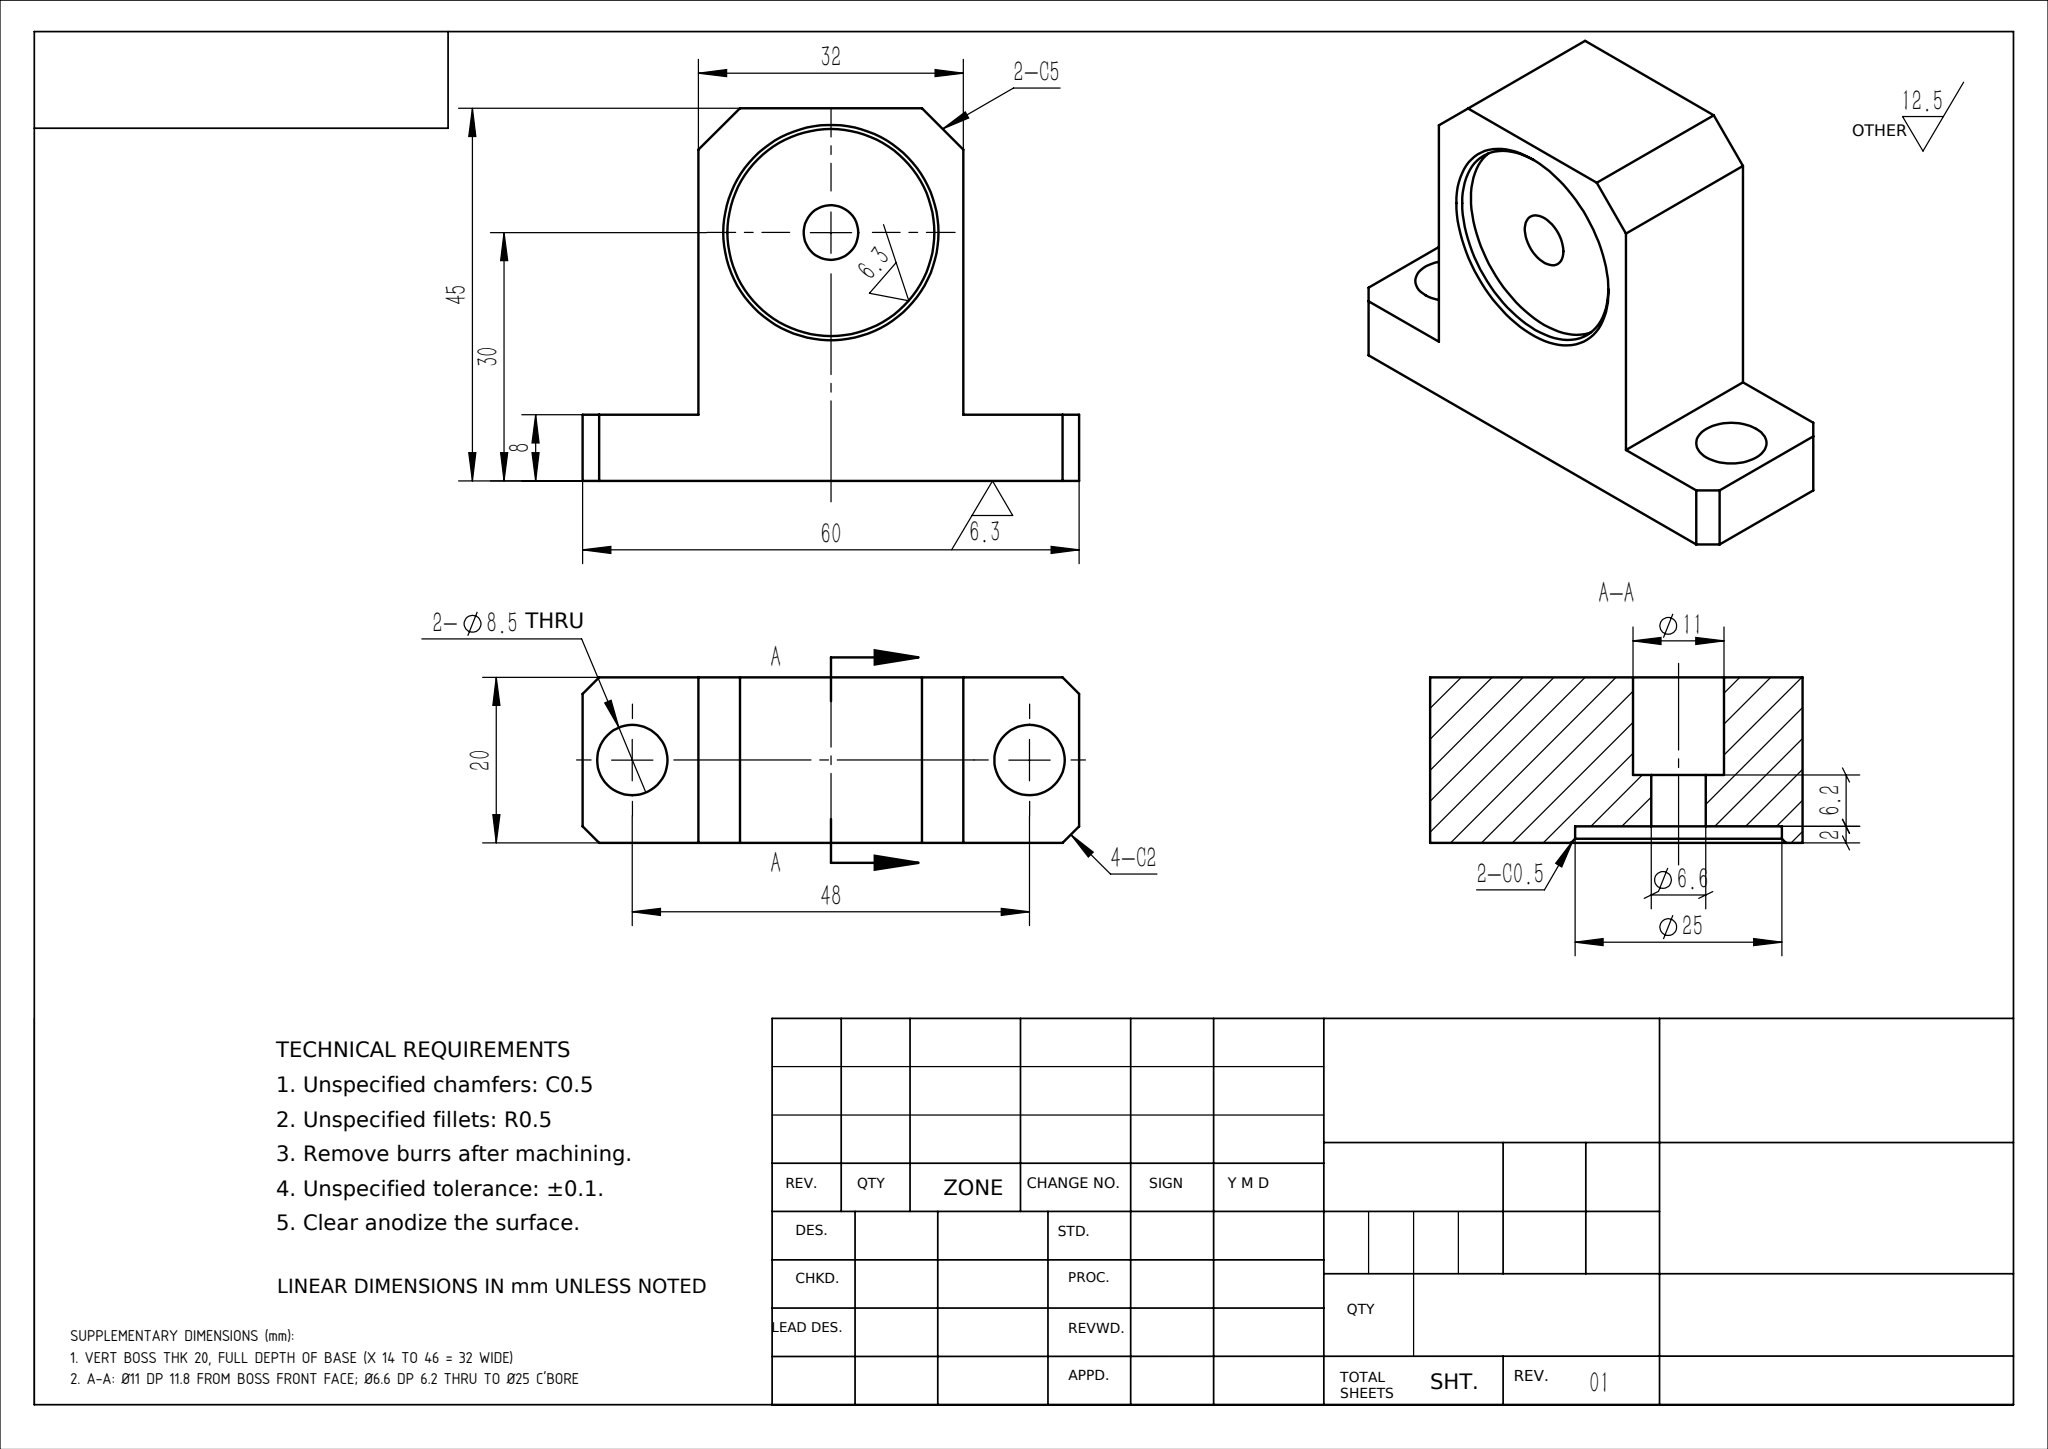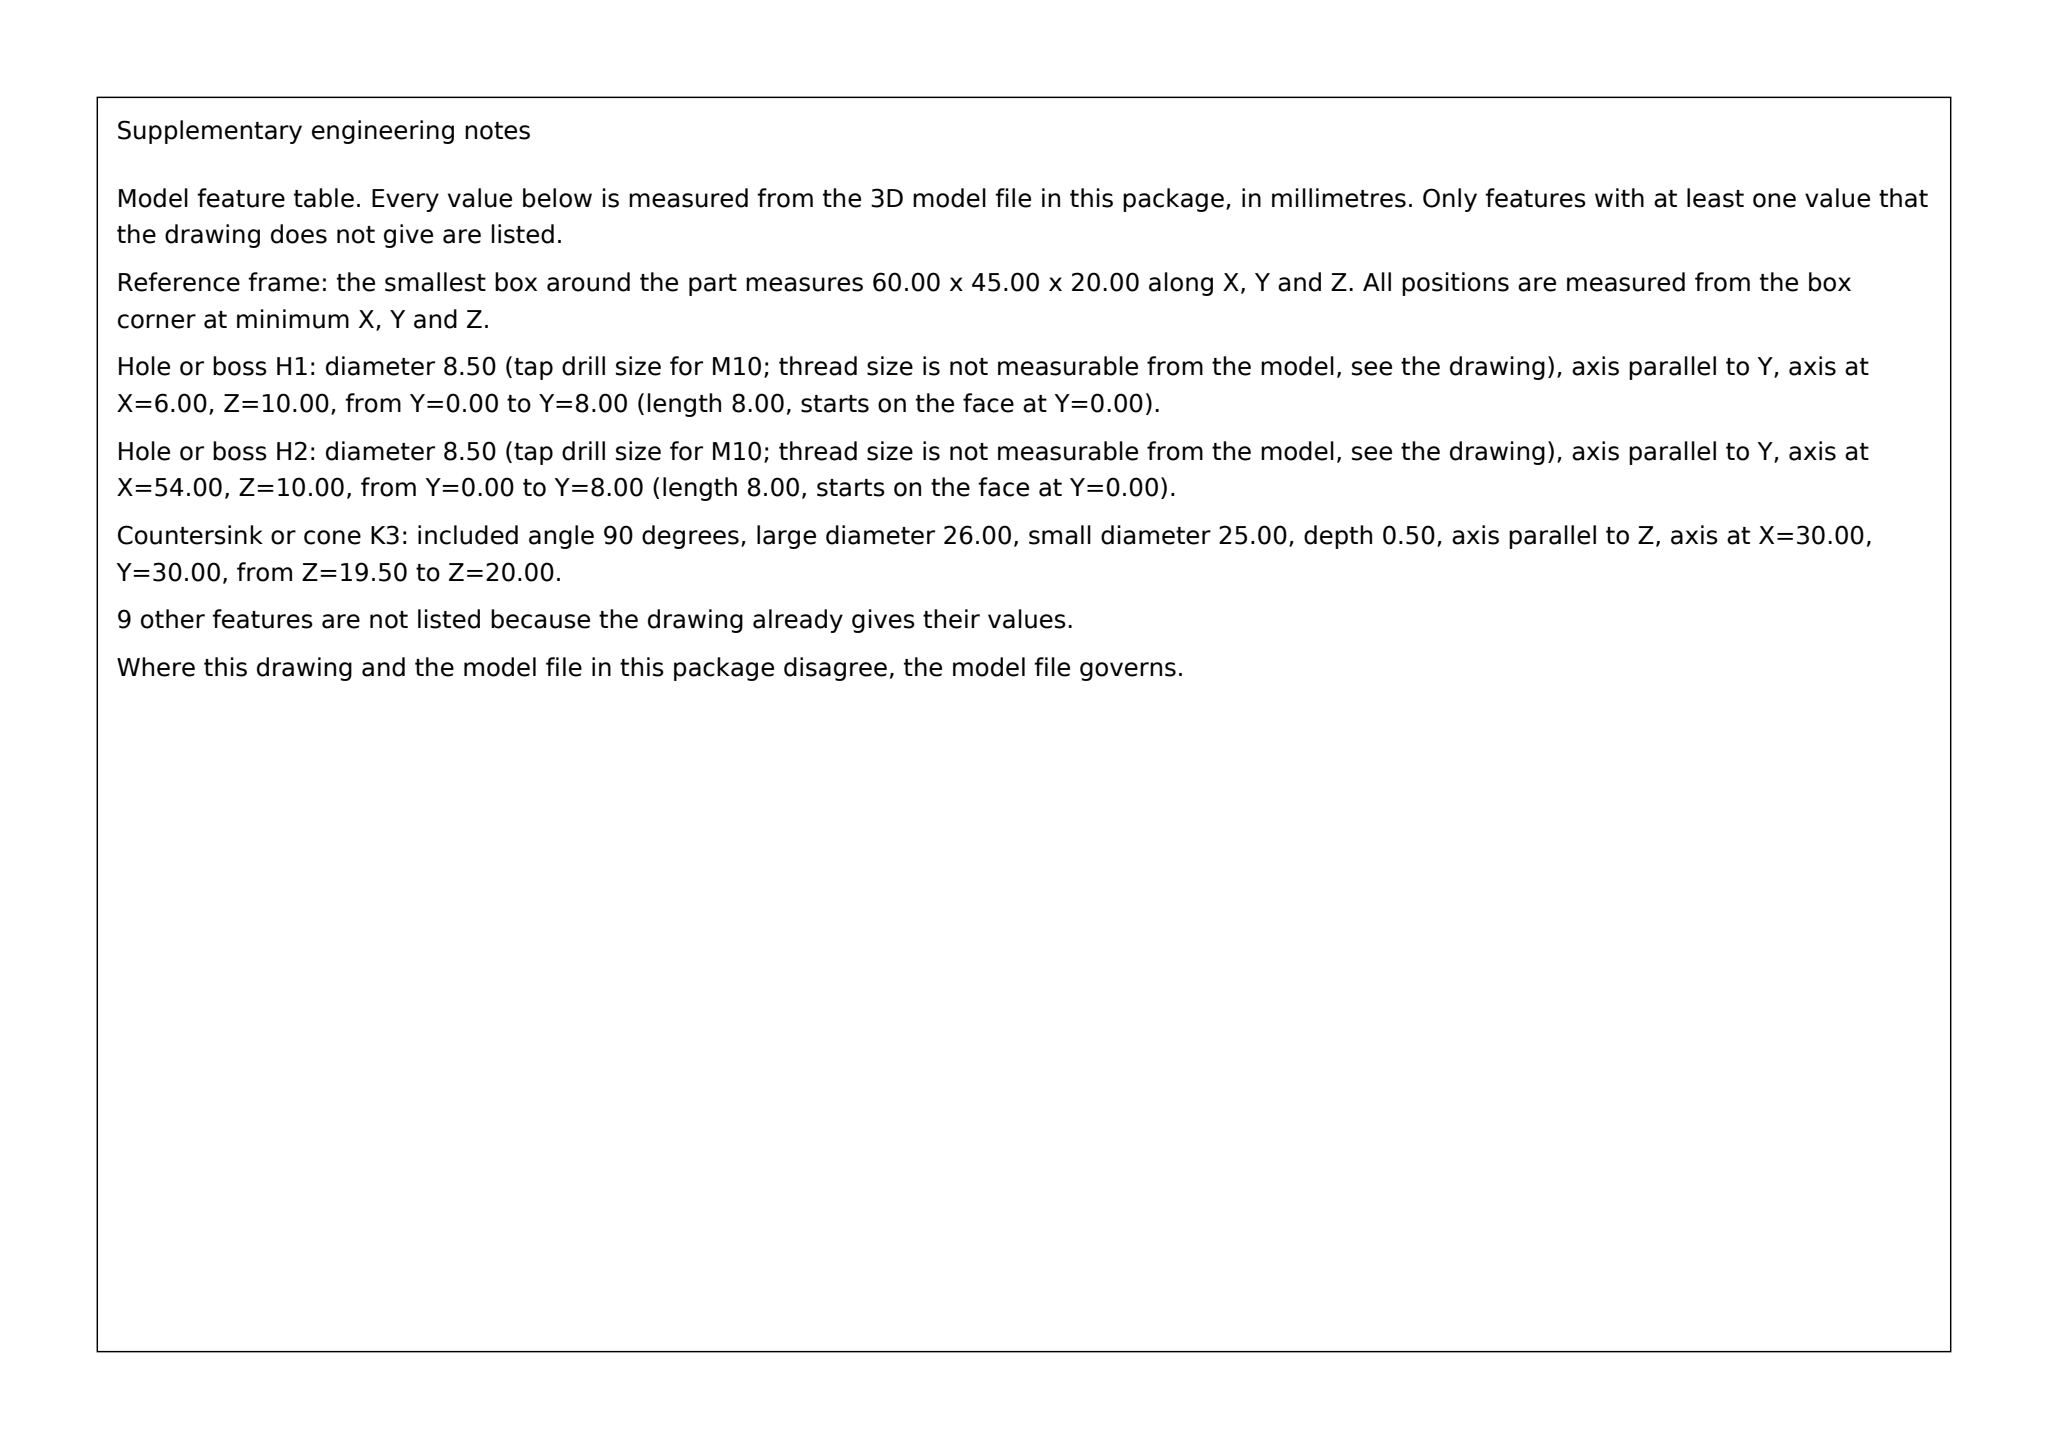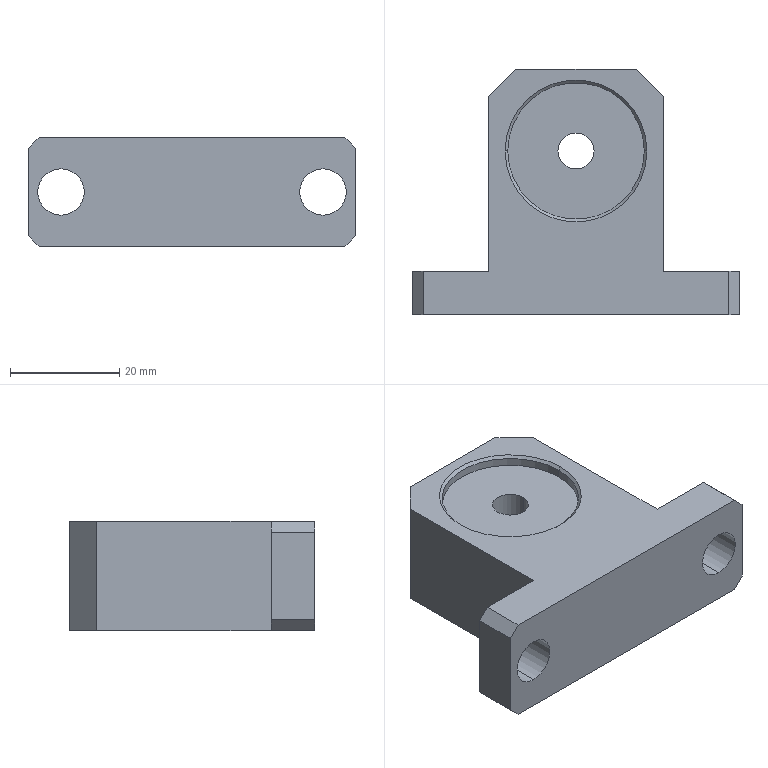Part | SolidWorks | mm | 1 solid | 30 faces | box 60 x 45 x 20 mm | volume 29483 mm3 | plane 18 | cylinder 10 | cone 2 | commonest cylinder face diameters 8.5 x4 11 x2 6.6 x2 25 x2
build123d program:
from build123d import *

# Parameters (mm, degrees)
BOSS_EXTRUDE1_DEPTH                               = 20
SKETCH2_R                                         = 12.5
CUT_EXTRUDE1_DEPTH                                = 2
CHAMFER1_SIZE                                     = 5
HOLE_SIZE_ACCORDING_TO_TYPE_1_OF_HEXA_D           = 6.6
HOLE_SIZE_ACCORDING_TO_TYPE_1_OF_HEXA_CBORE_D     = 11
HOLE_SIZE_ACCORDING_TO_TYPE_1_OF_HEXA_CBORE_DEPTH = 11.8
CHAMFER2_SIZE                                     = 0.5
SKETCH5_R                                         = 4.25
CUT_EXTRUDE2_DEPTH                                = 52.662
CHAMFER3_SIZE                                     = 2


with BuildPart() as part:
    # Sketch1 → Boss-Extrude1 (new body)
    with BuildSketch(Plane.XY):
        Polygon((-30, 0), (30, 0), (30, 8), (16, 8), (16, 45), (-16, 45), (-16, 8), (-30, 8), align=None)
    extrude(amount=BOSS_EXTRUDE1_DEPTH)

    # Sketch2 → Cut-Extrude1 (cut)
    with BuildSketch(Plane.XY.offset(20)):
        with Locations((0, 30)):
            Circle(SKETCH2_R)
    extrude(amount=-CUT_EXTRUDE1_DEPTH, mode=Mode.SUBTRACT)

    # Chamfer1
    chamfer1_edges = [part.edges().sort_by_distance(p)[0] for p in [
        (-16, 45, 10),
        (16, 45, 10),
    ]]
    chamfer(chamfer1_edges, length=CHAMFER1_SIZE)

    # Hole Size _ according to_ type 1 of Hexa (through all)
    with Locations(Plane(origin=(0, 0, 0), x_dir=(-1, 0, 0), z_dir=(0, 0, -1))):
        with Locations((0, 30)):
            CounterBoreHole(HOLE_SIZE_ACCORDING_TO_TYPE_1_OF_HEXA_D / 2, HOLE_SIZE_ACCORDING_TO_TYPE_1_OF_HEXA_CBORE_D / 2, HOLE_SIZE_ACCORDING_TO_TYPE_1_OF_HEXA_CBORE_DEPTH)

    # Chamfer2
    chamfer2_edges = [part.edges().sort_by_distance(p)[0] for p in [
        (-12.5, 30, 20),
    ]]
    chamfer(chamfer2_edges, length=CHAMFER2_SIZE)

    # Sketch5 → Cut-Extrude2 (cut, through all)
    with BuildSketch(Plane(origin=(0, 8, 0), x_dir=(1, 0, 0), z_dir=(0, 1, 0))):
        with Locations(Location((-24, -10, 0), (0, 0, 270))):
            Circle(SKETCH5_R)
        with Locations(Location((24, -10, 0), (0, 0, 90))):
            Circle(SKETCH5_R)
    extrude(amount=-CUT_EXTRUDE2_DEPTH, mode=Mode.SUBTRACT)

    # Chamfer3
    chamfer3_edges = [part.edges().sort_by_distance(p)[0] for p in [
        (30, 4, 20),
        (-30, 4, 0),
        (-30, 4, 20),
        (30, 4, 0),
    ]]
    chamfer(chamfer3_edges, length=CHAMFER3_SIZE)


solid = part.part